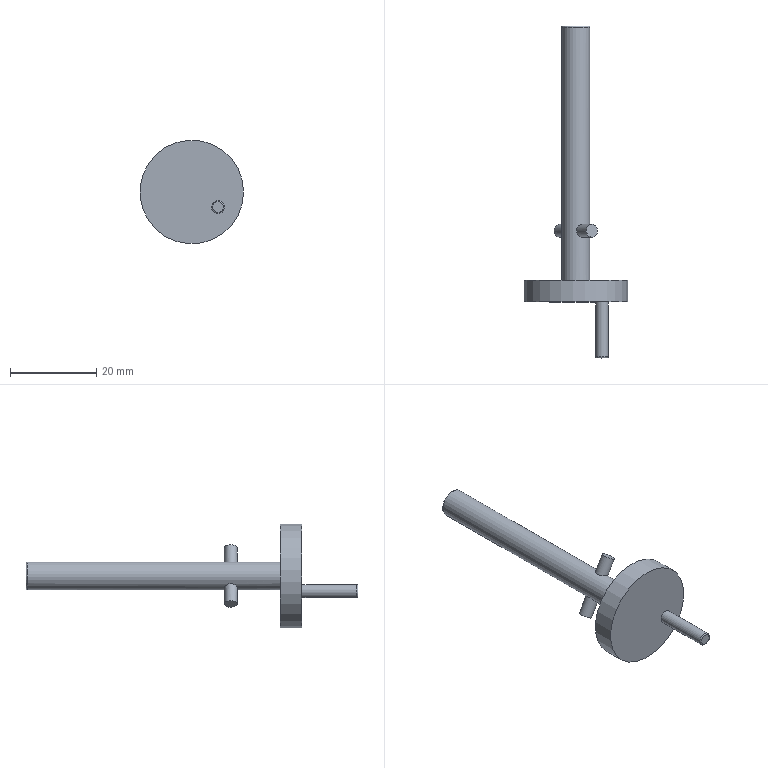Component | NX | CRANKSHAFT | 1 solid | 13 faces | volume 4373 mm3 | plane 6 | cylinder 5 | torus 2 | commonest cylinder face diameters 3 x3 6.5 x1 24 x1